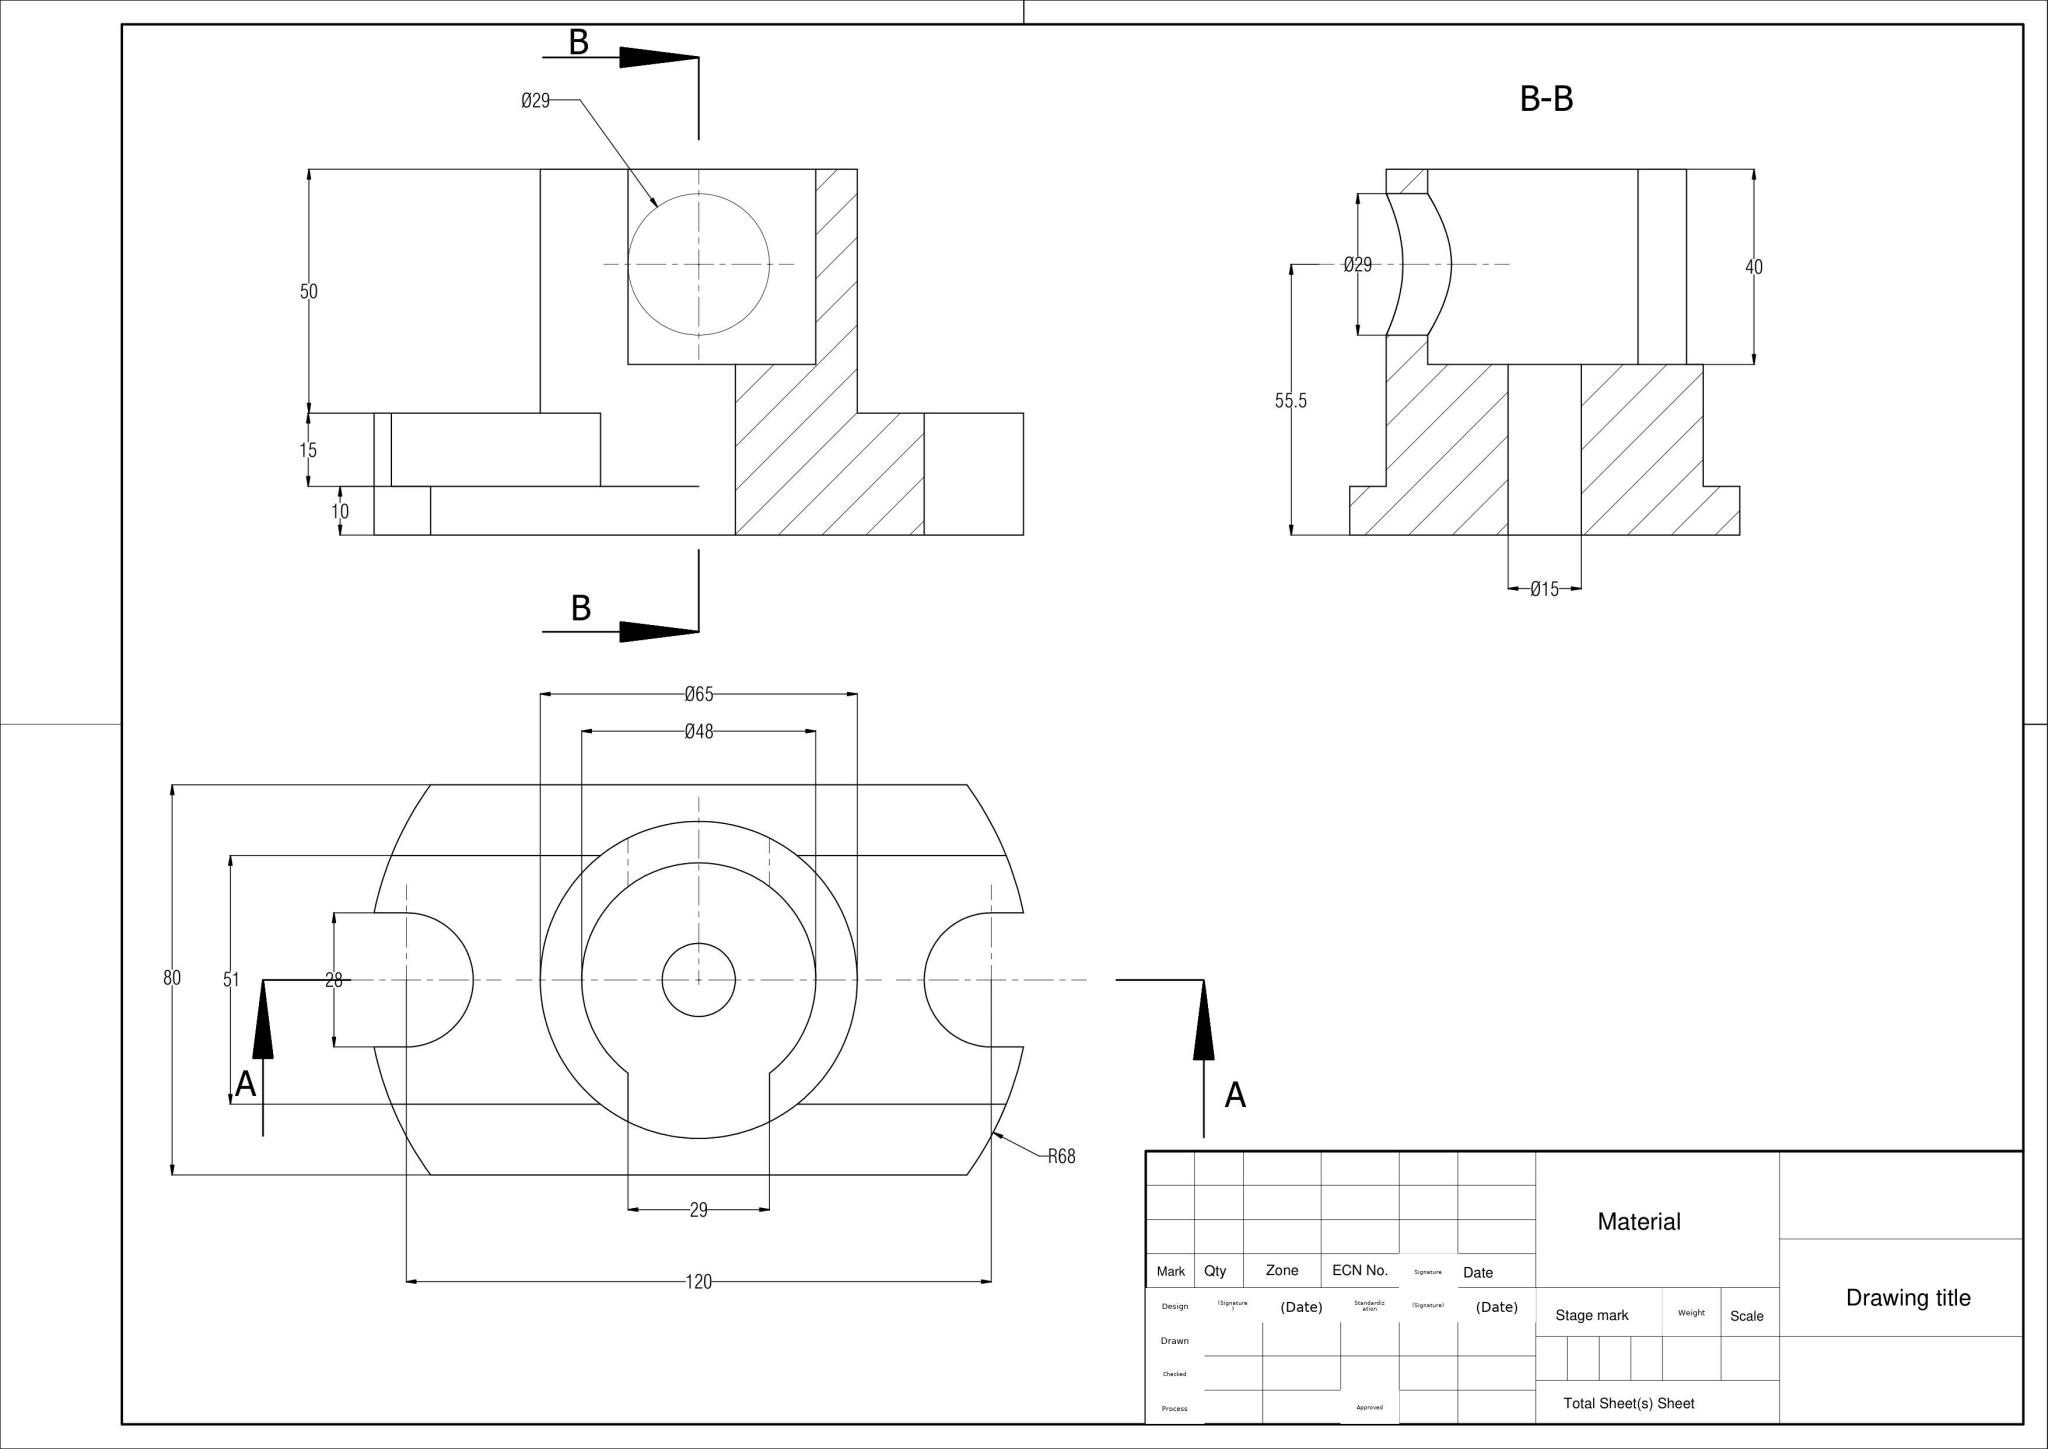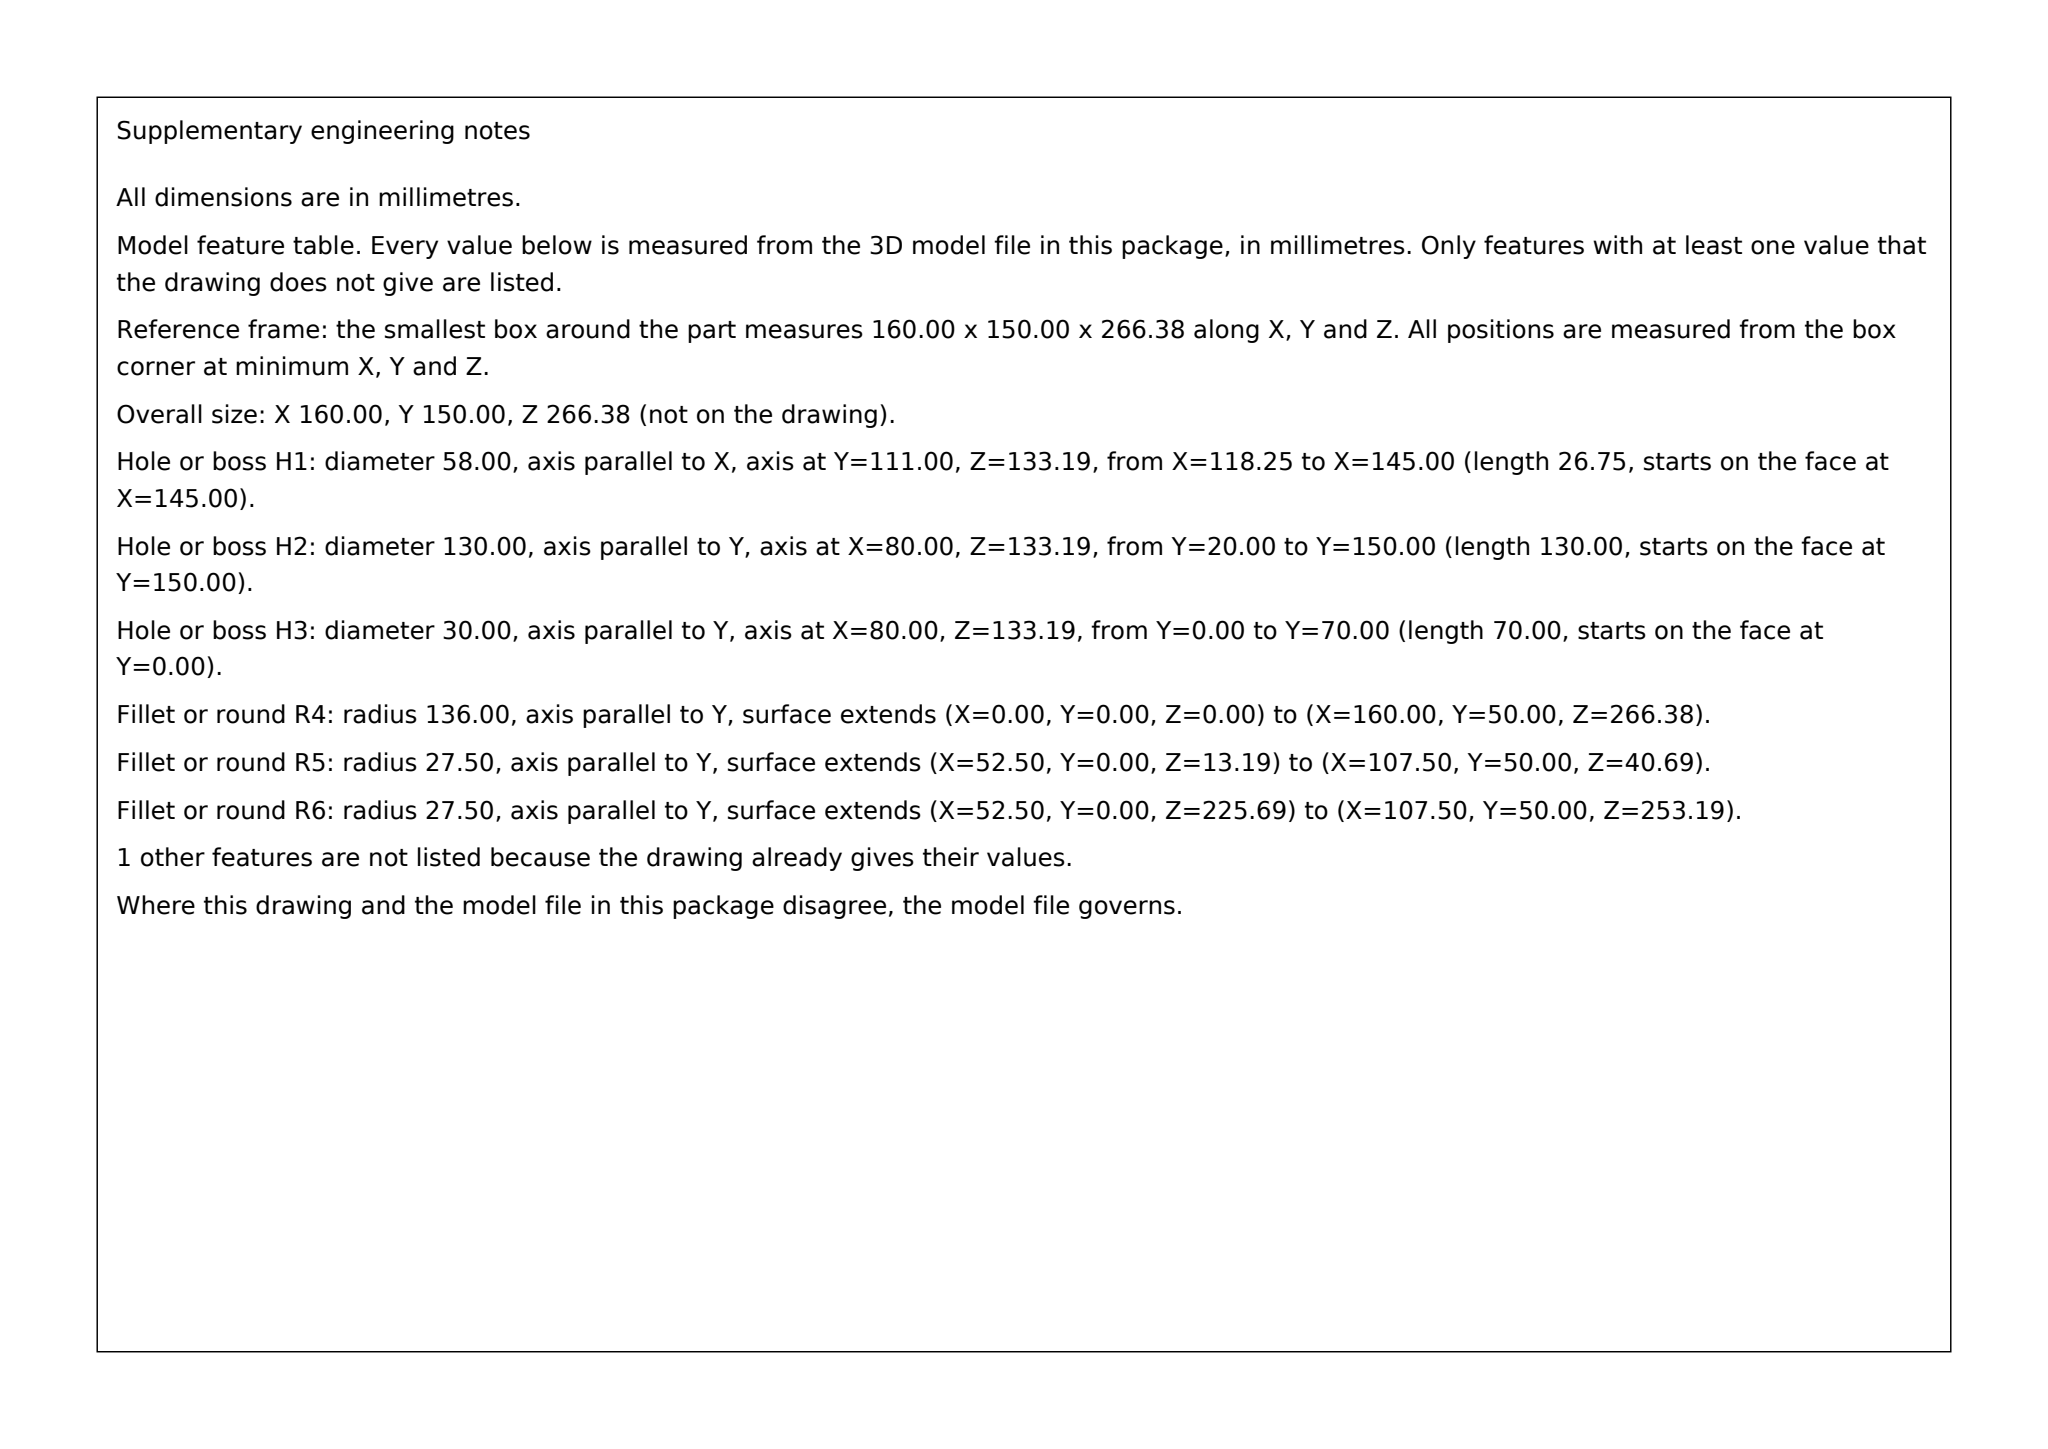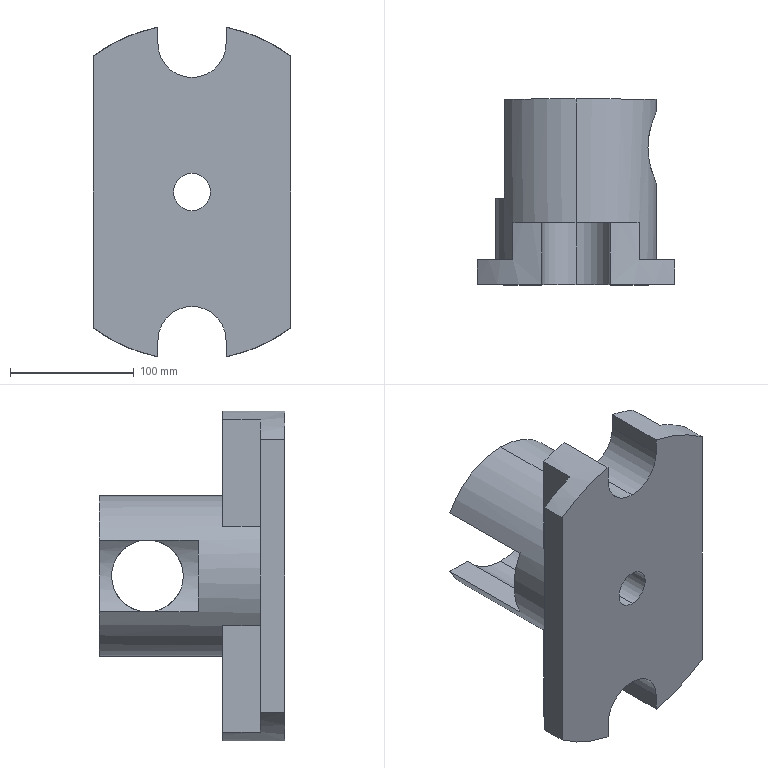Part | SolidWorks | mm | 1 solid | 35 faces | box 160 x 150 x 266.38 mm | volume 2043345 mm3 | plane 19 | cylinder 16 | commonest cylinder face diameters 272 x4 96 x3 55 x3 130 x2 58 x2 30 x2